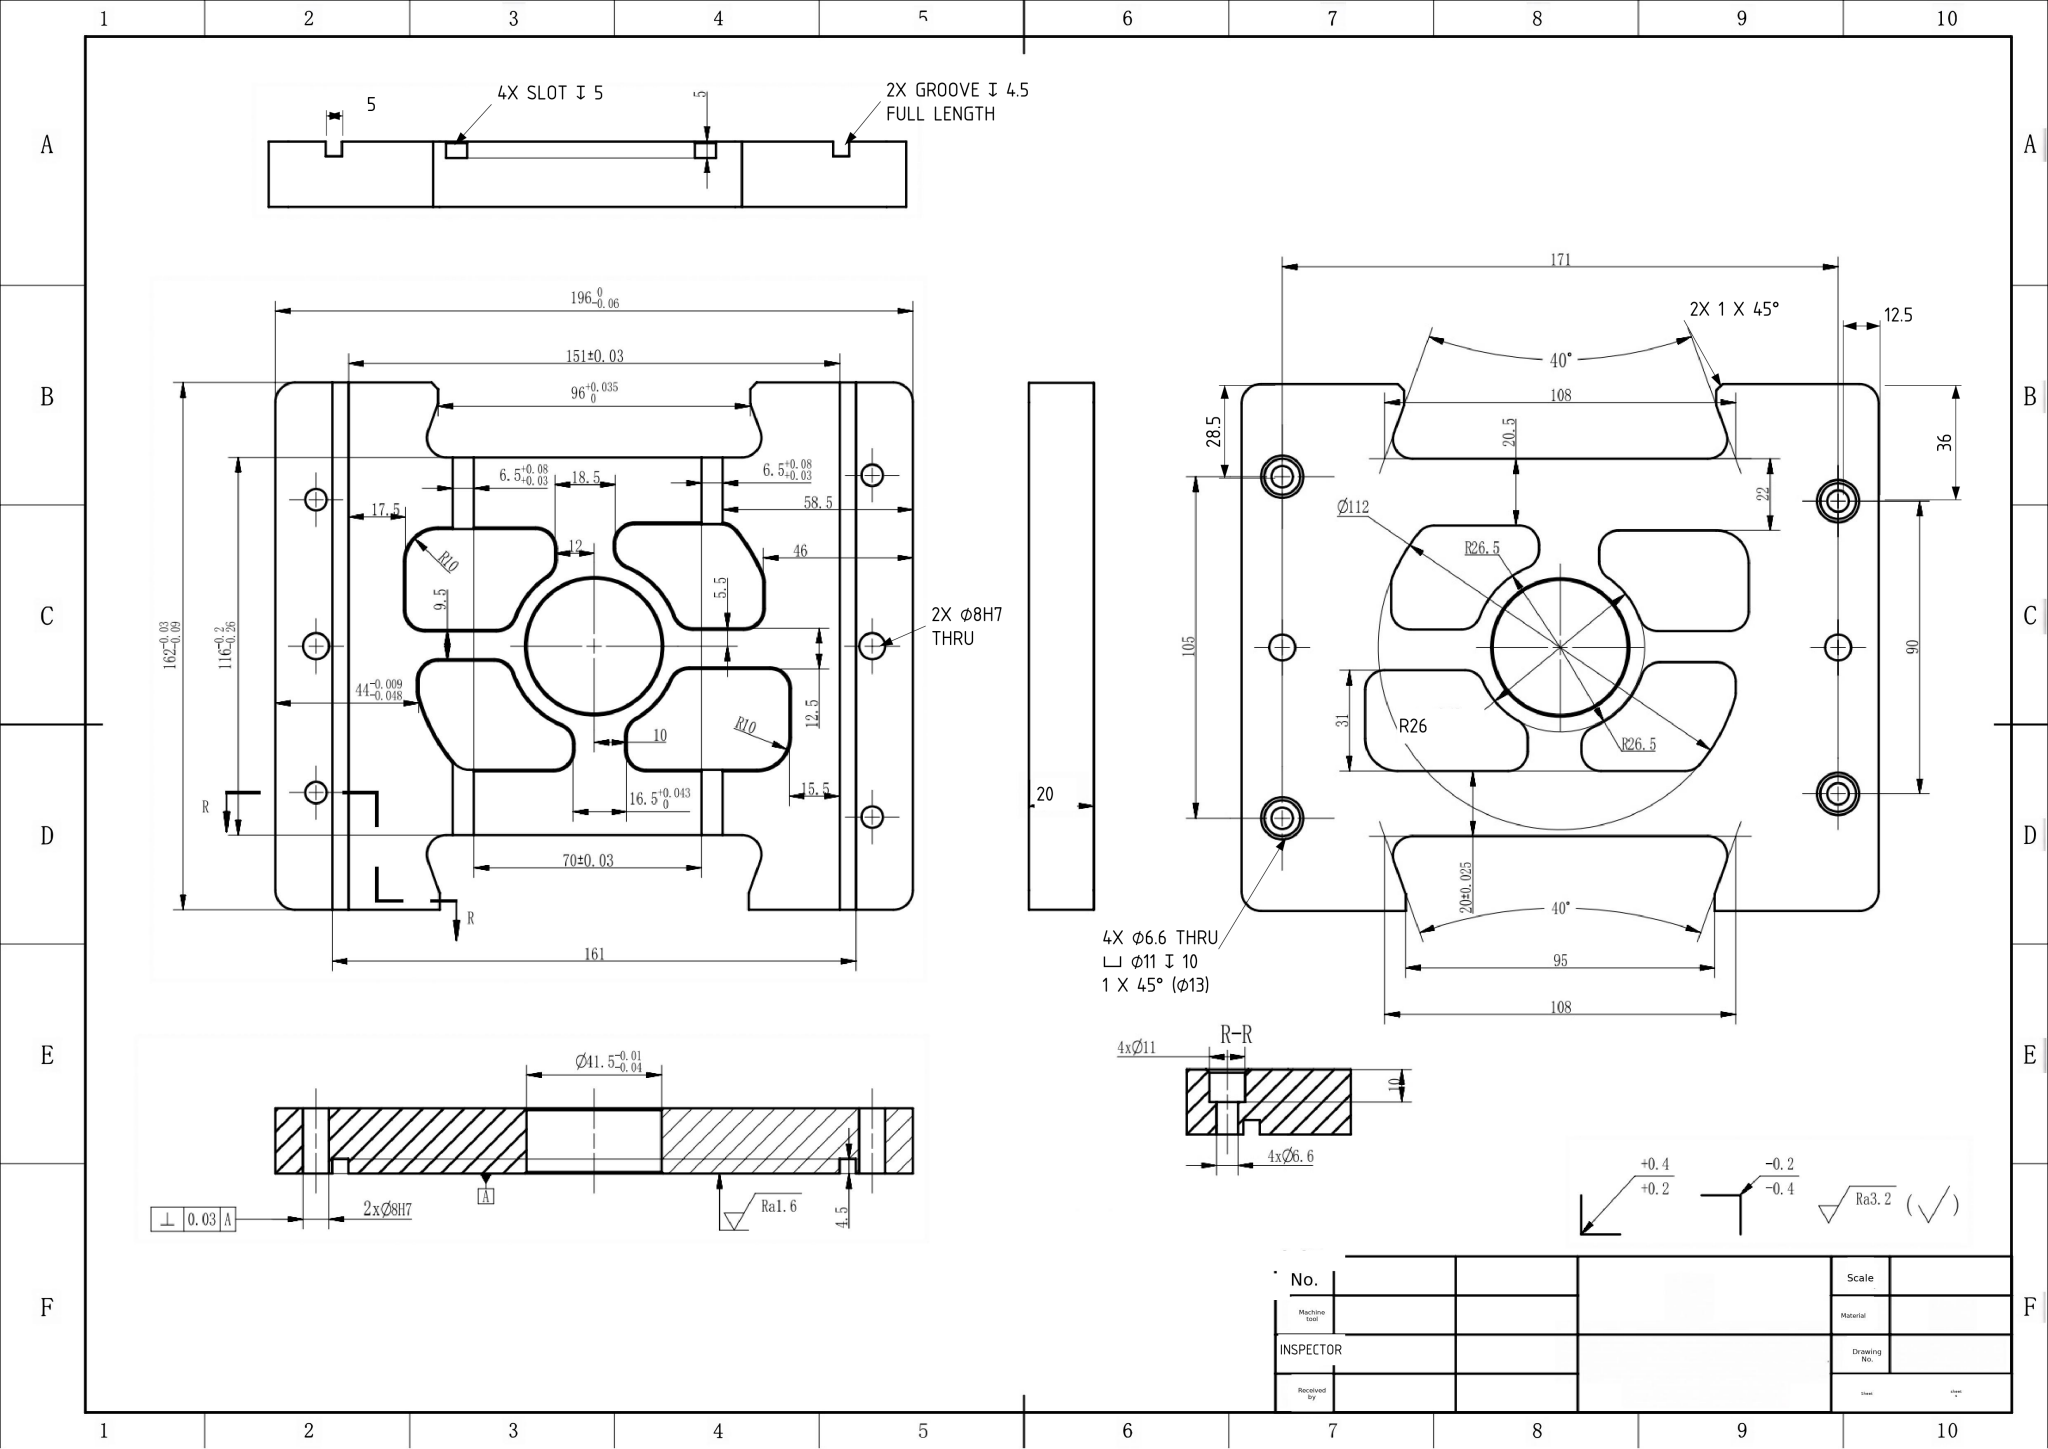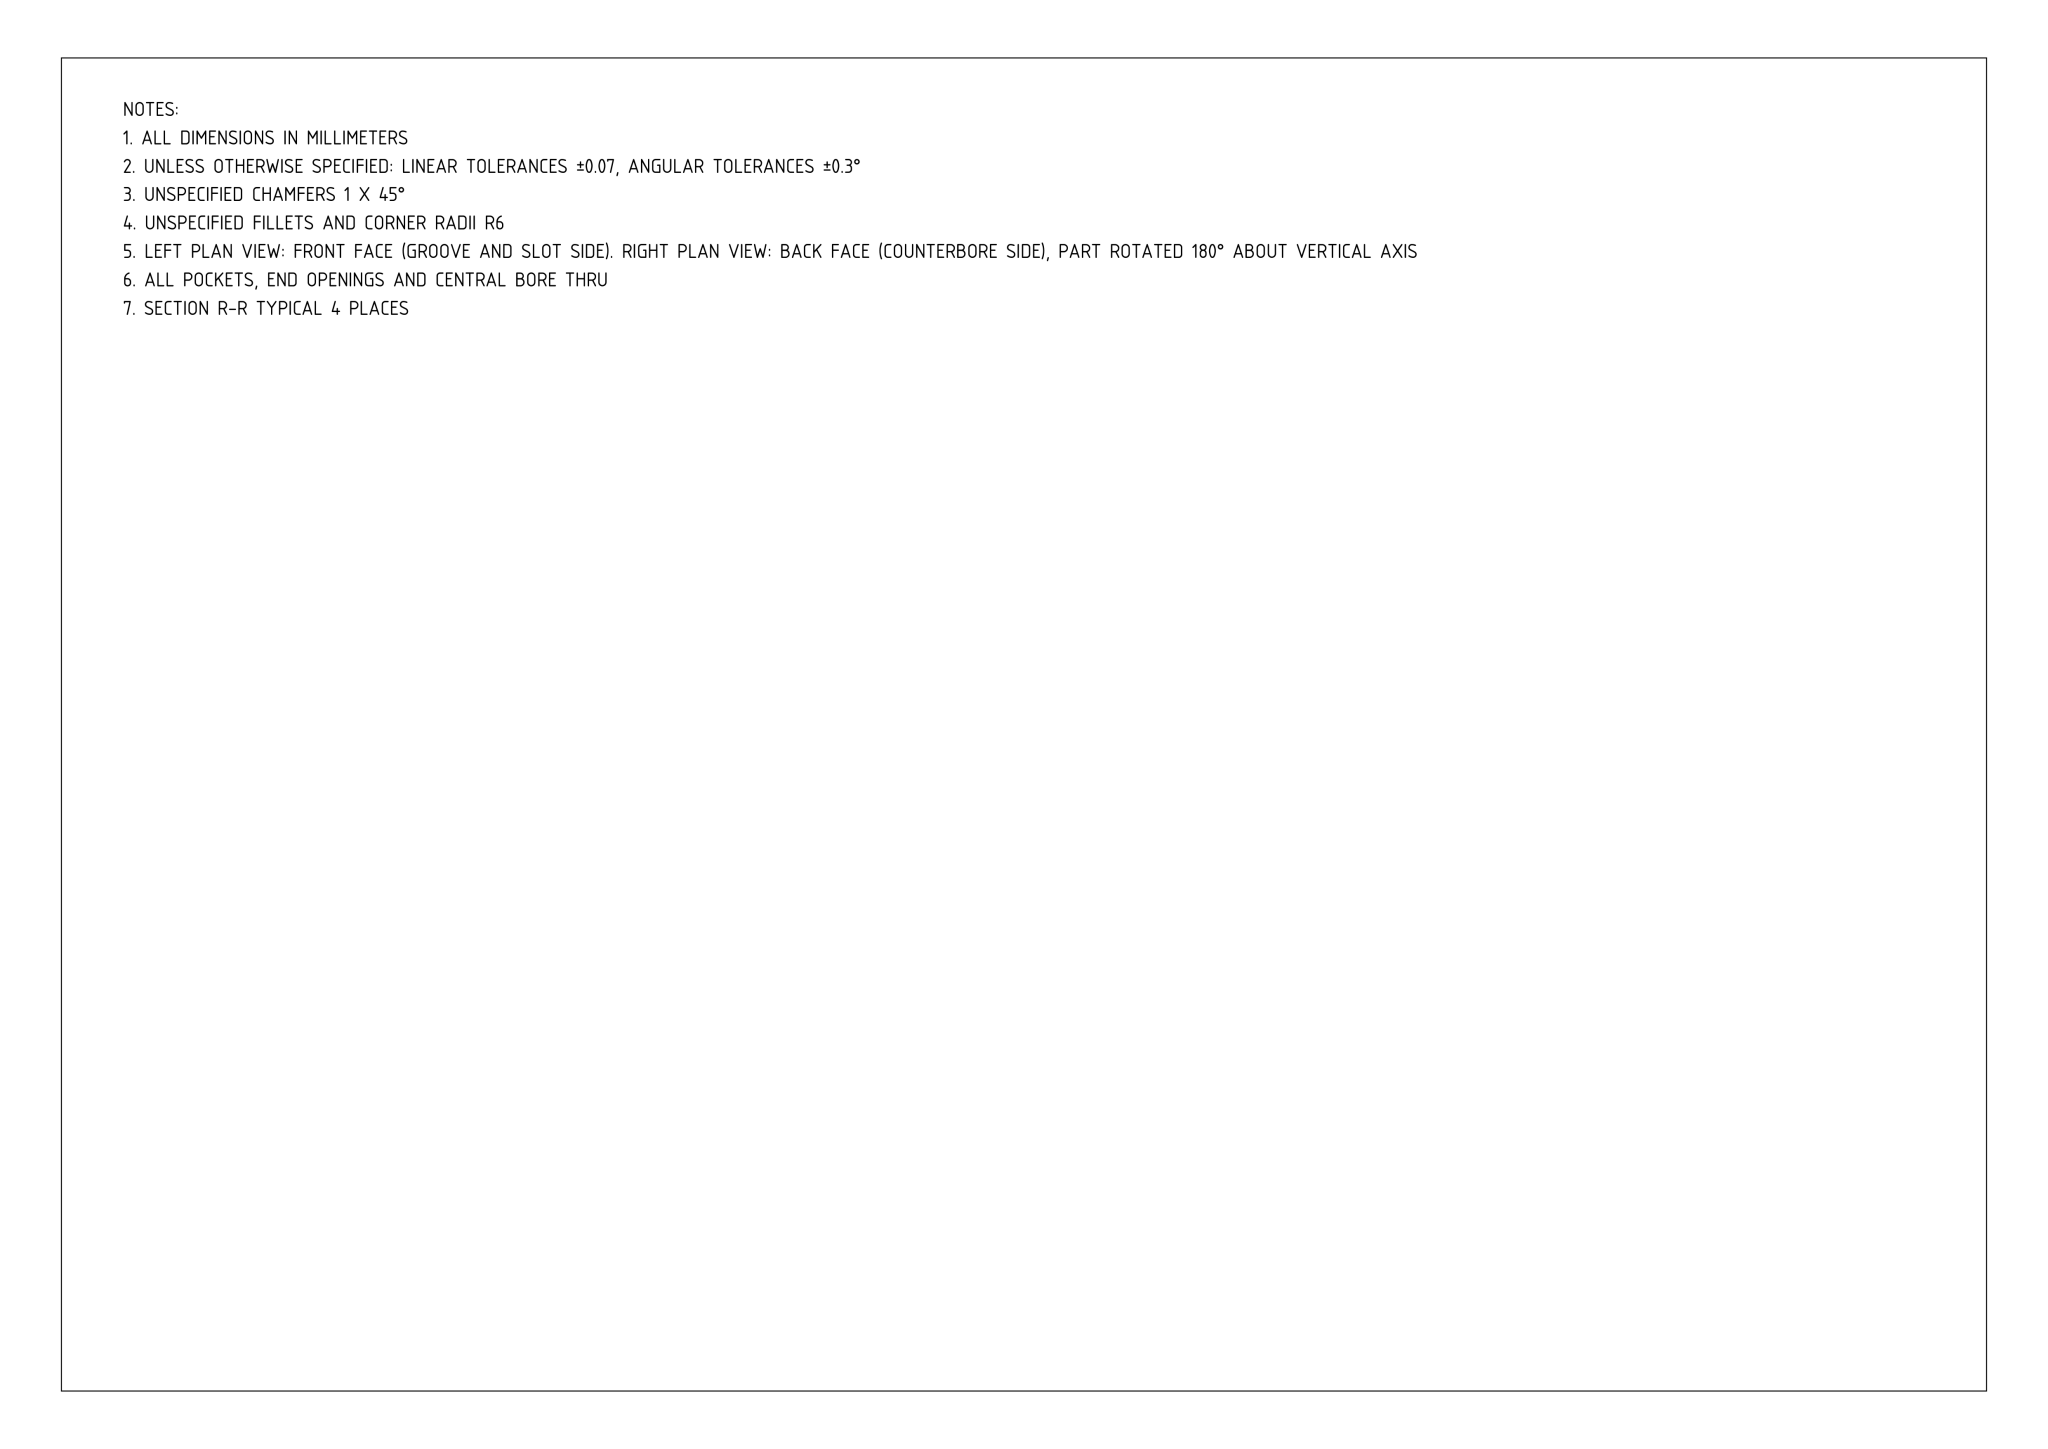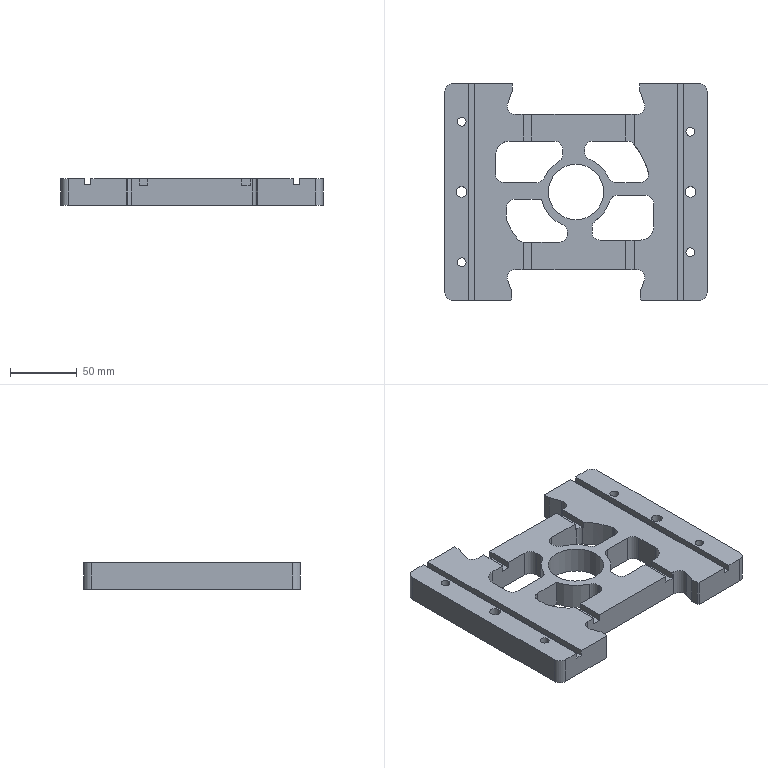Part | NX | mm | 1 solid | 110 faces | box 196 x 162 x 20 mm | volume 402959 mm3 | plane 60 | cylinder 46 | cone 4 | commonest cylinder face diameters 12 x27 6.6 x4 11 x4 52 x2 53 x2 112 x2 20 x2 8 x2